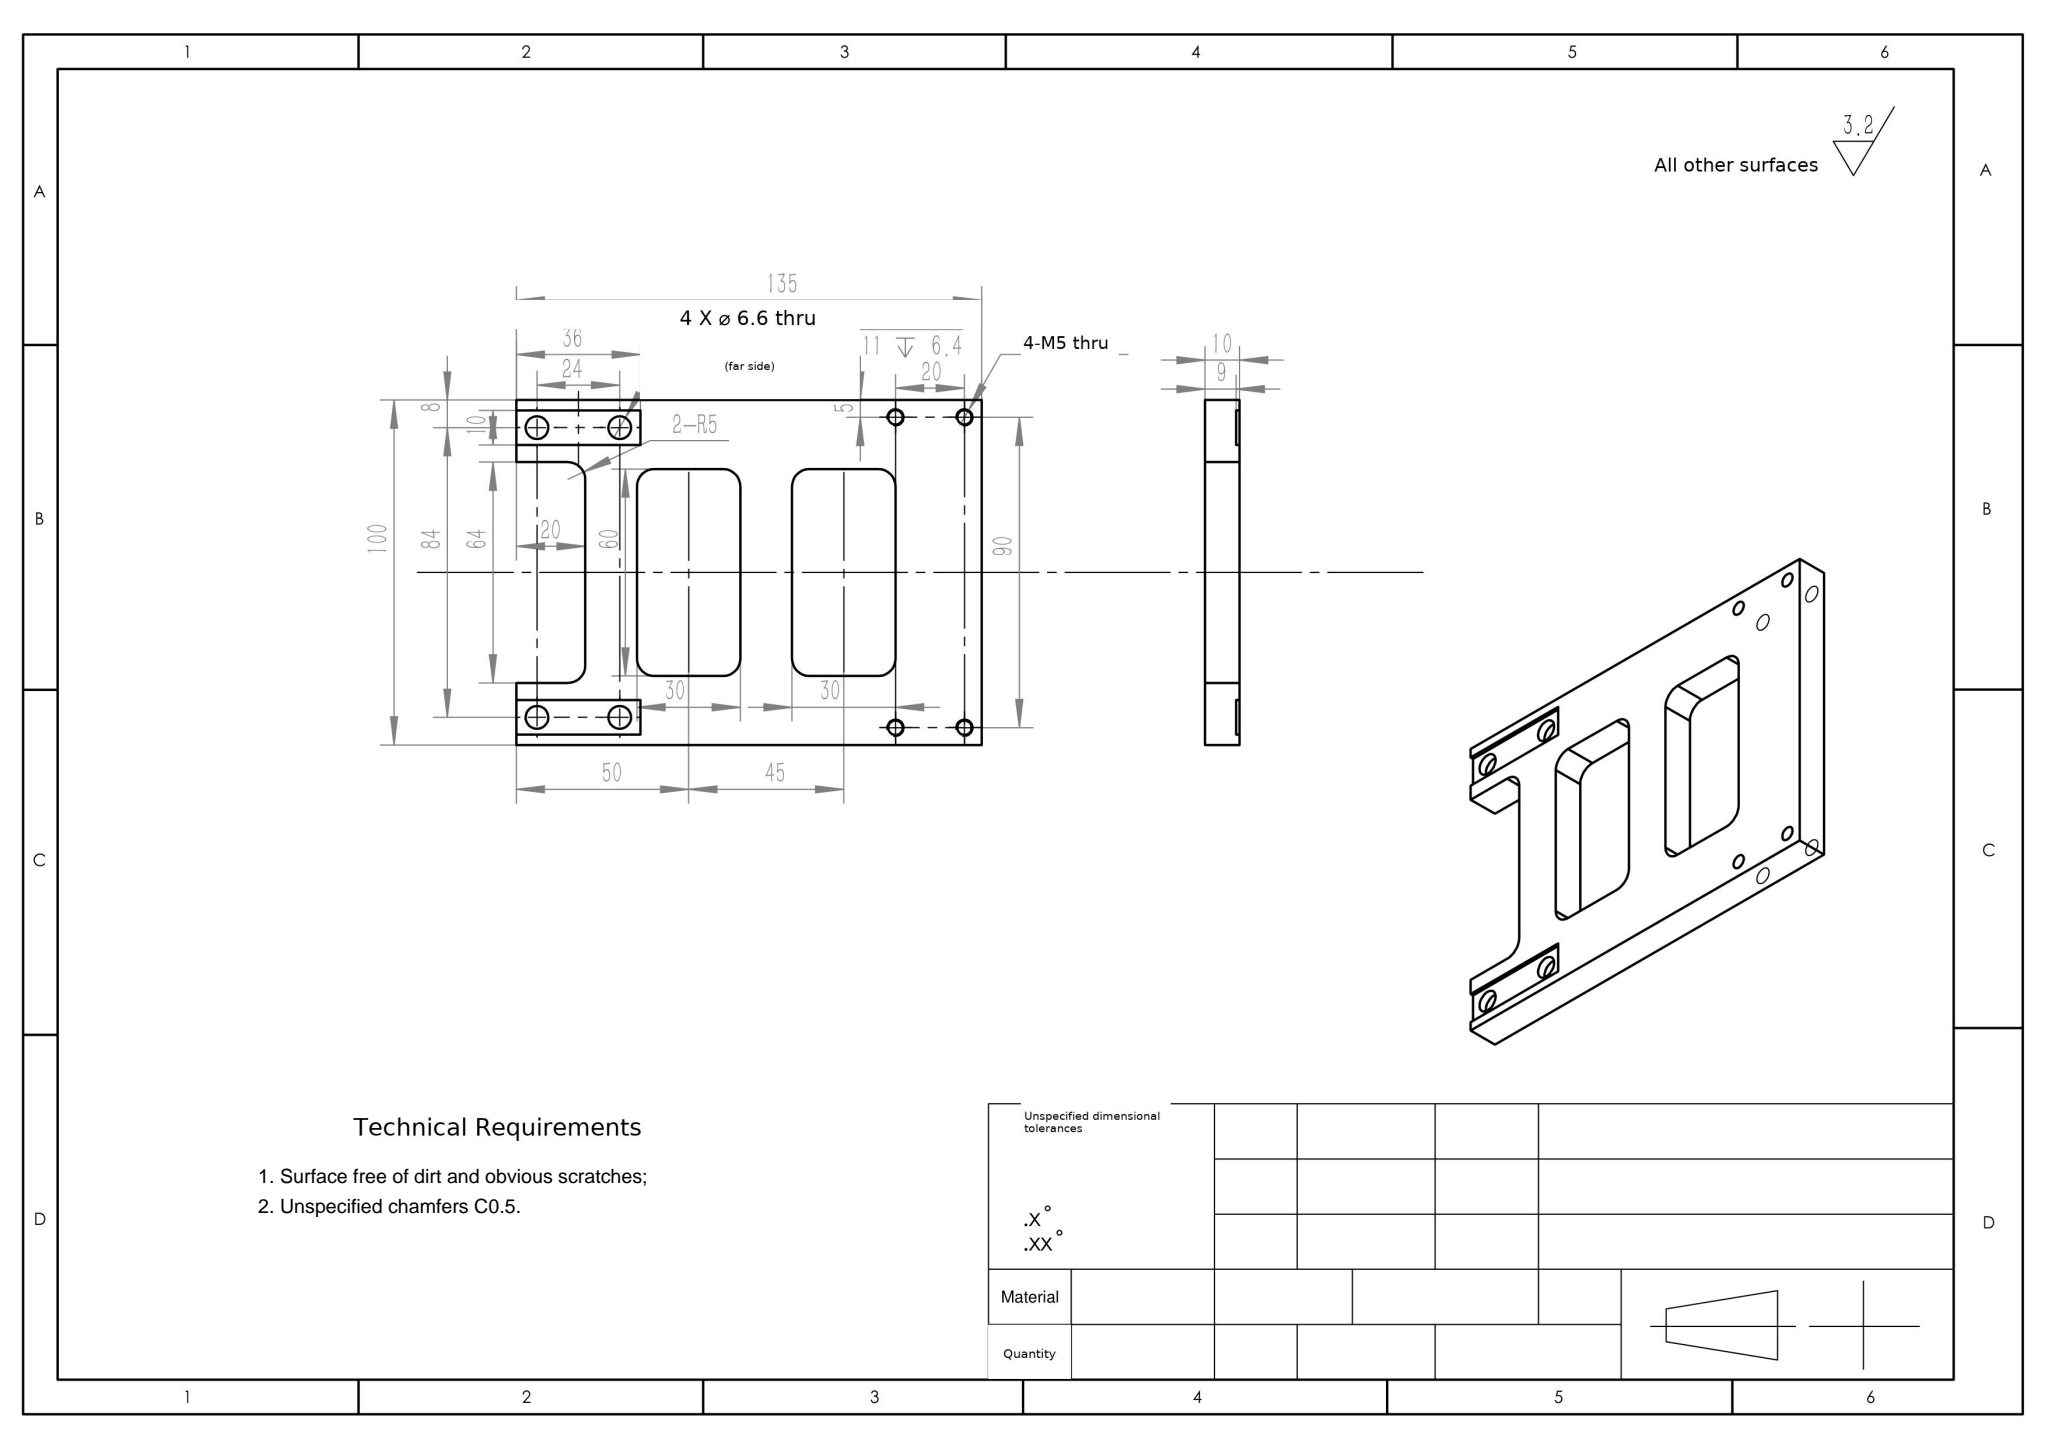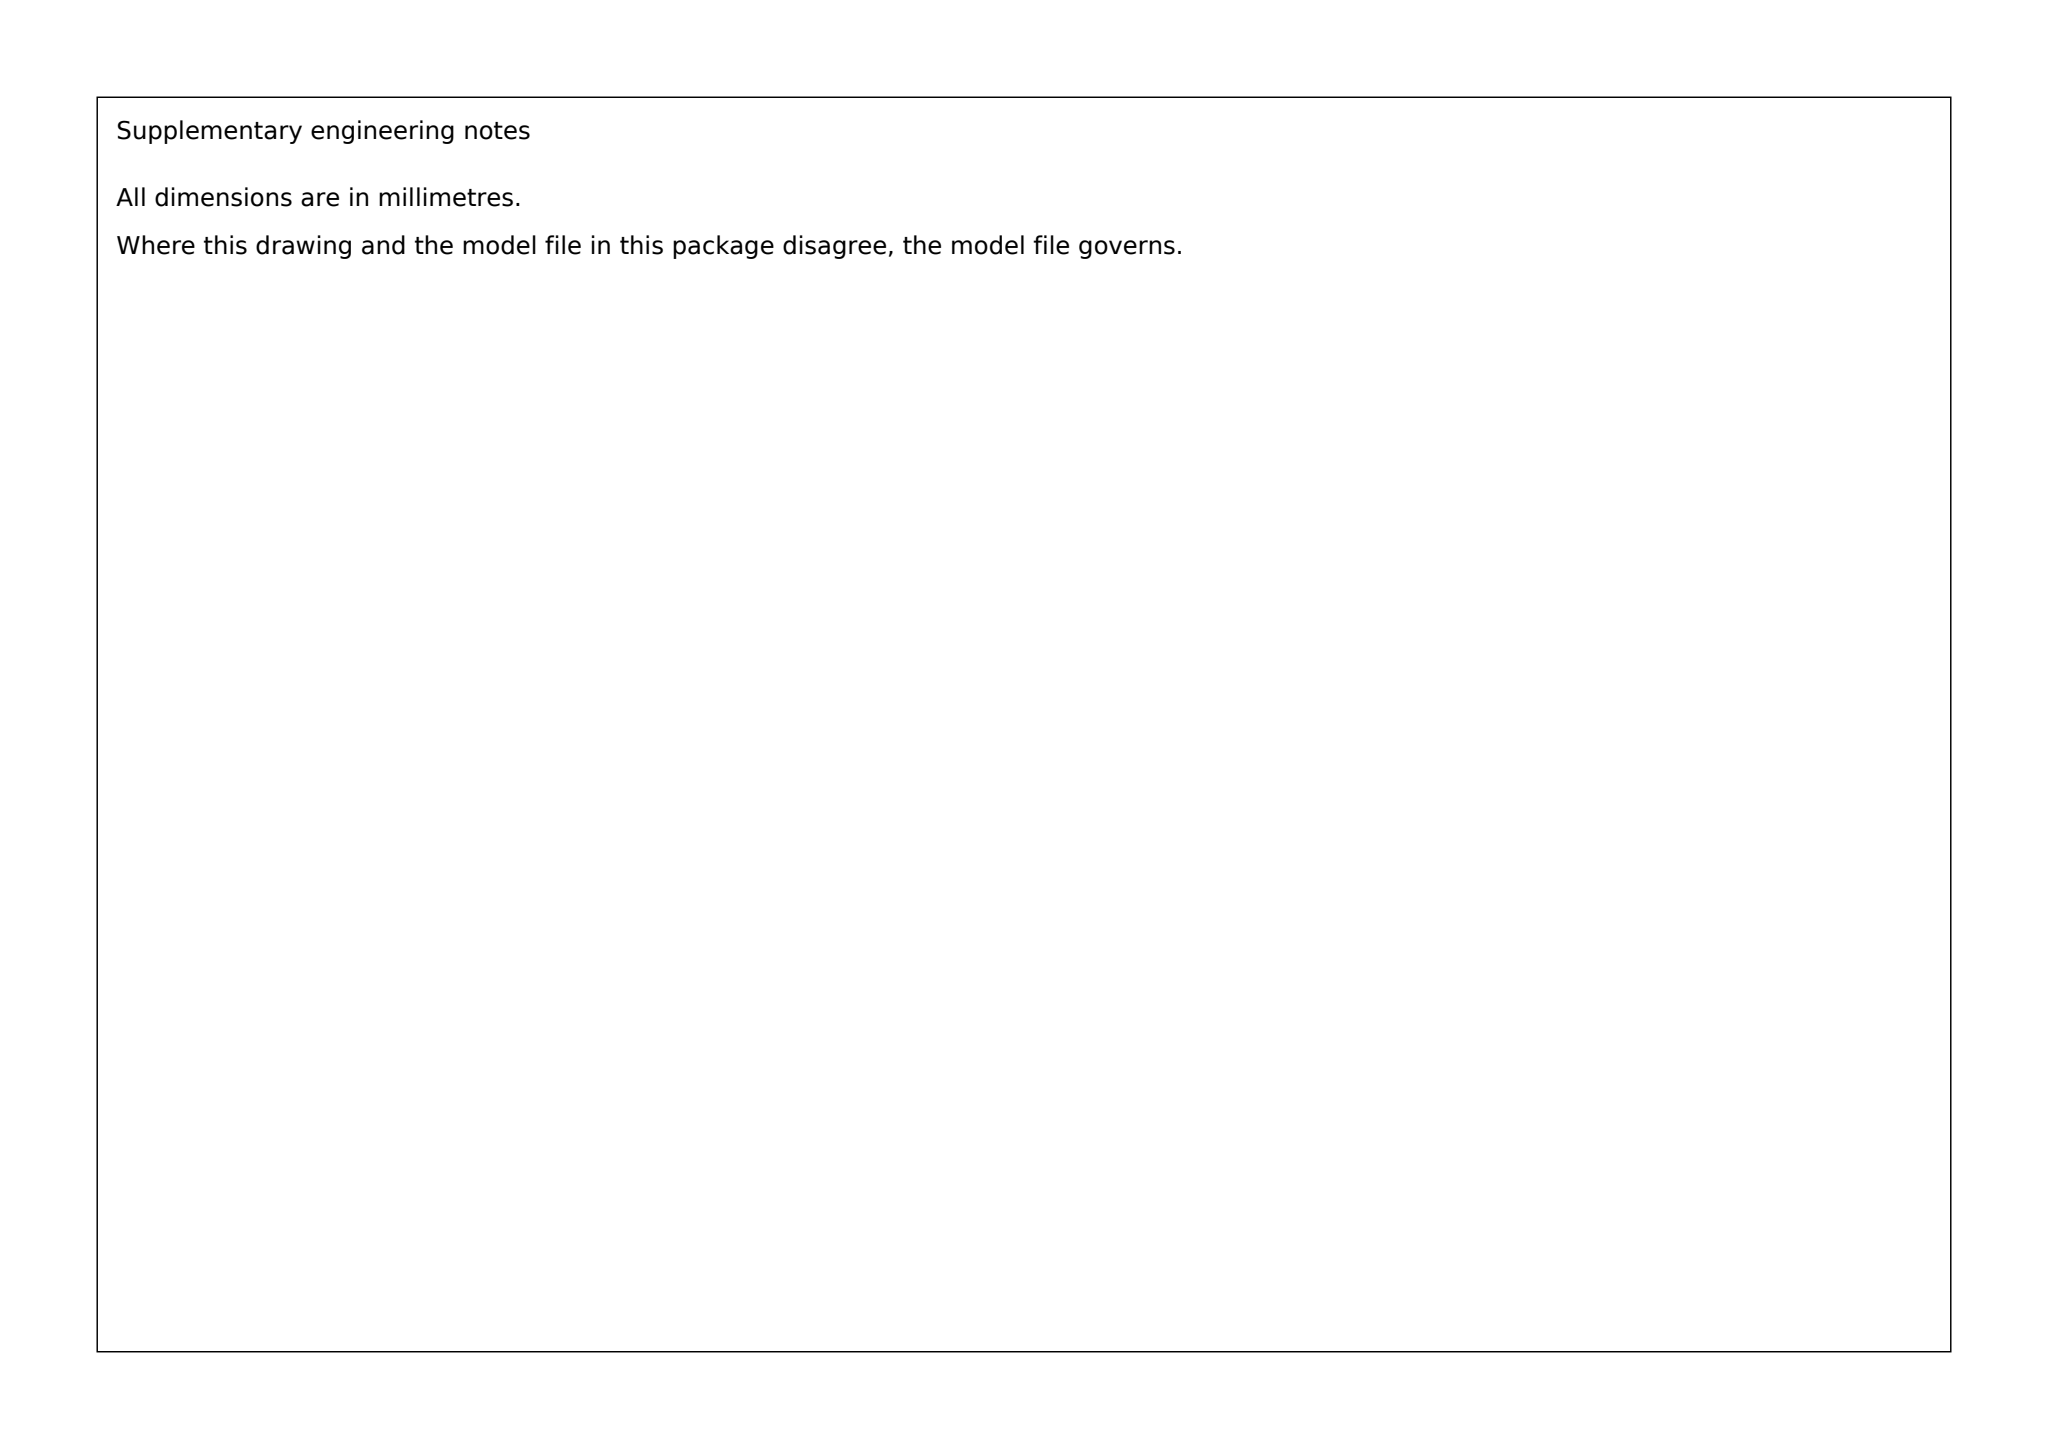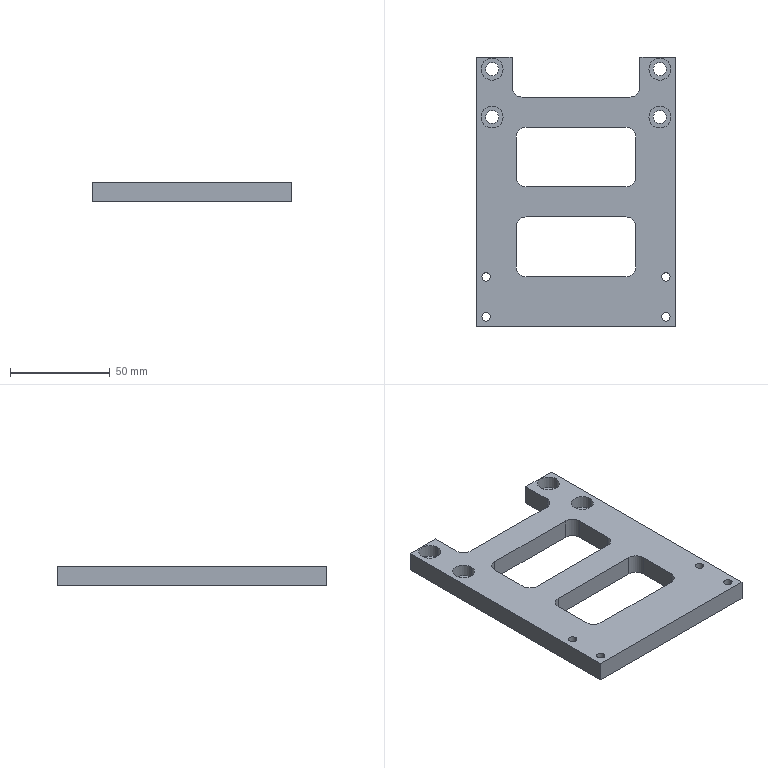Part | SolidWorks | mm | 1 solid | 64 faces | box 100 x 135 x 10 mm | volume 82674 mm3 | cylinder 34 | plane 30 | commonest cylinder face diameters 10 x10 4.2 x8 11 x8 6.6 x8
build123d program:
from build123d import *

# Parameters (mm, degrees)
SKETCH1_W                                       = 100
SKETCH1_H                                       = 135
BOSS_EXTRUDE1_DEPTH                             = 10
SKETCH2_W                                       = 10
SKETCH2_H                                       = 36
CUT_EXTRUDE1_DEPTH                              = 1
M6_HEX_SOCKET_HEAD_CAP_SCREW_CBORE1_D           = 6.6
M6_HEX_SOCKET_HEAD_CAP_SCREW_CBORE1_CBORE_D     = 11
M6_HEX_SOCKET_HEAD_CAP_SCREW_CBORE1_CBORE_DEPTH = 6.4
CUT_EXTRUDE2_REACH                              = 86.595
SKETCH6_W                                       = 64
SKETCH6_H                                       = 20
CUT_EXTRUDE3_REACH                              = 86.595
SKETCH7_W                                       = 60
SKETCH7_H                                       = 30
FILLET1_R                                       = 5
M5_TAPPED_HOLE1_D                               = 4.2


with BuildPart() as part:
    # Sketch1 → Boss-Extrude1 (new body)
    with BuildSketch(Plane.XY):
        Rectangle(SKETCH1_W, SKETCH1_H)
    extrude(amount=BOSS_EXTRUDE1_DEPTH)

    # Sketch2 → Cut-Extrude1 (cut)
    with BuildSketch(Plane(origin=(0, 0, 0), x_dir=(-1, 0, 0), z_dir=(0, 0, -1))):
        with Locations((-42, 49.5)):
            Rectangle(SKETCH2_W, SKETCH2_H)
        with Locations((42, 49.5)):
            Rectangle(SKETCH2_W, SKETCH2_H)
    extrude(amount=-CUT_EXTRUDE1_DEPTH, mode=Mode.SUBTRACT)

    # M6 Hex Socket Head Cap Screw CBORE1 (through all)
    with Locations(Plane.XY.offset(10)):
        with Locations((42, 61.5), (42, 37.5), (-42, 37.5), (-42, 61.5)):
            CounterBoreHole(M6_HEX_SOCKET_HEAD_CAP_SCREW_CBORE1_D / 2, M6_HEX_SOCKET_HEAD_CAP_SCREW_CBORE1_CBORE_D / 2, M6_HEX_SOCKET_HEAD_CAP_SCREW_CBORE1_CBORE_DEPTH)

    # Sketch6 → Cut-Extrude2 (cut, up to next)
    with BuildSketch(Plane.XY.offset(10), mode=Mode.PRIVATE) as cut_extrude2_sk1:
        with Locations((0, 57.5)):
            Rectangle(SKETCH6_W, SKETCH6_H)
    cut_extrude2_tool1 = extrude(cut_extrude2_sk1.sketch, amount=-CUT_EXTRUDE2_REACH, mode=Mode.PRIVATE) & part.part
    add(cut_extrude2_tool1.solids().sort_by_distance((0, 57.5, 10))[0], mode=Mode.SUBTRACT)

    # Sketch7 → Cut-Extrude3 (cut, up to next)
    with BuildSketch(Plane.XY.offset(10), mode=Mode.PRIVATE) as cut_extrude3_sk1:
        with Locations((0, 17.5)):
            Rectangle(SKETCH7_W, SKETCH7_H)
    cut_extrude3_tool1 = extrude(cut_extrude3_sk1.sketch, amount=-CUT_EXTRUDE3_REACH, mode=Mode.PRIVATE) & part.part
    # Sketch7 → Cut-Extrude3 (cut, up to next)
    with BuildSketch(Plane.XY.offset(10), mode=Mode.PRIVATE) as cut_extrude3_sk2:
        with Locations((0, -27.5)):
            Rectangle(SKETCH7_W, SKETCH7_H)
    cut_extrude3_tool2 = extrude(cut_extrude3_sk2.sketch, amount=-CUT_EXTRUDE3_REACH, mode=Mode.PRIVATE) & part.part
    add(cut_extrude3_tool1.solids().sort_by_distance((0, 17.5, 10))[0], mode=Mode.SUBTRACT)
    add(cut_extrude3_tool2.solids().sort_by_distance((0, -27.5, 10))[0], mode=Mode.SUBTRACT)

    # Fillet1
    fillet1_edges = [part.edges().sort_by_distance(p)[0] for p in [
        (30, -12.5, 5),
        (30, -42.5, 5),
        (-30, -42.5, 5),
        (-30, -12.5, 5),
        (32, 47.5, 5),
        (-32, 47.5, 5),
        (30, 32.5, 5),
        (30, 2.5, 5),
        (-30, 2.5, 5),
        (-30, 32.5, 5),
    ]]
    fillet(fillet1_edges, radius=FILLET1_R)

    # M5 Tapped Hole1 (through all)
    with Locations(Plane.XY.offset(10)):
        with Locations((-45, -42.5), (-45, -62.5), (45, -62.5), (45, -42.5)):
            Hole(M5_TAPPED_HOLE1_D / 2)


solid = part.part